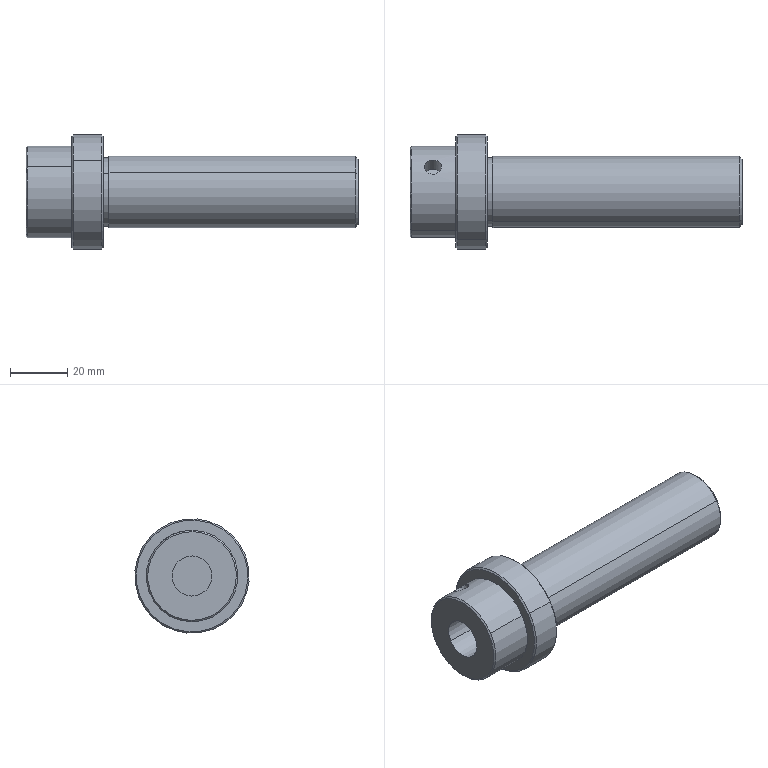Component | SolidWorks | 4-12-12ClampingAxisAssembly-1_4-12-3ClampingAxis-1 | 1 solid | 27 faces | box 116 x 40 x 40 mm | volume 68513 mm3 | cylinder 12 | cone 8 | plane 7 | commonest cylinder face diameters 6 x2 40 x2 32 x2 14 x2 25 x2 24 x2
build123d program:
from build123d import *

# Parameters (mm, degrees)
CHAMFER1_SIZE      = 1
CHAMFER2_SIZE      = 0.5
SKETCH2_R          = 3
CUT_EXTRUDE1_DEPTH = 6


with BuildPart() as part:
    # Sketch1 → Revolve1 (revolve)
    with BuildSketch(Plane(origin=(0, 0, 0), x_dir=(0, 0, -1), z_dir=(1, 0, 0)), mode=Mode.PRIVATE) as revolve1_sk:
        Polygon((0, 7), (0, 16), (16, 16), (16, 20), (27, 20), (27, 12), (29, 12), (29, 12.5), (116, 12.5), (116, 0), (10, 0), (10, 7), align=None)
    revolve(revolve1_sk.sketch.rotate(Axis((0, 0, 0), (0, 0, -1)), 90), axis=Axis((0, 0, 0), (0, 0, -1)))

    # Chamfer1
    chamfer1_edges = [part.edges().sort_by_distance(p)[0] for p in [
        (-12.5, 0, -116),
    ]]
    chamfer(chamfer1_edges, length=CHAMFER1_SIZE)

    # Chamfer2
    chamfer2_edges = [part.edges().sort_by_distance(p)[0] for p in [
        (-20, 0, -27),
        (-20, 0, -16),
        (-16, 0, 0),
    ]]
    chamfer(chamfer2_edges, length=CHAMFER2_SIZE)

    # Sketch2 → Cut-Extrude1 (cut)
    with BuildSketch(Plane(origin=(0, 16, 0), x_dir=(-1, 0, 0), z_dir=(0, 1, 0))):
        with Locations(Location((0, -8, 0), (0, 0, 90))):
            Circle(SKETCH2_R)
    extrude(amount=-CUT_EXTRUDE1_DEPTH, mode=Mode.SUBTRACT)


solid = part.part

# Placed as in the assembly
solid = solid.moved(Location((-152.809, -4.181, 0), (-166.184, -90, 137.125)))
STEP:
#1=COLOUR_RGB('',0.7922,0.8196,0.9333);
#2=FILL_AREA_STYLE_COLOUR('',#1);
#3=FILL_AREA_STYLE('',(#2));
#4=SURFACE_STYLE_FILL_AREA(#3);
#5=SURFACE_SIDE_STYLE('',(#4));
#6=SURFACE_STYLE_USAGE(.BOTH.,#5);
#7=PRESENTATION_STYLE_ASSIGNMENT((#6));
#8=CARTESIAN_POINT('',(-5.583,0.05163,0.329));
#9=VERTEX_POINT('',#8);
#10=CARTESIAN_POINT('',(-5.819,0.05163,0.329));
#11=VERTEX_POINT('',#10);
#12=CARTESIAN_POINT('',(-5.701,0.05163,0.329));
#13=DIRECTION('',(-0.,0.5492,0.8357));
#14=DIRECTION('',(-1.,-0.,0.));
#15=AXIS2_PLACEMENT_3D('',#12,#13,#14);
#16=CIRCLE('',#15,0.1181);
#17=EDGE_CURVE('',#9,#11,#16,.T.);
#18=ORIENTED_EDGE('',*,*,#17,.F.);
#19=CARTESIAN_POINT('',(-5.583,0.1814,0.5264));
#20=VERTEX_POINT('',#19);
#21=CARTESIAN_POINT('',(-5.583,0.05163,0.329));
#22=DIRECTION('',(-0.,0.5492,0.8357));
#23=VECTOR('',#22,39.37);
#24=LINE('',#21,#23);
#25=EDGE_CURVE('',#9,#20,#24,.T.);
#26=ORIENTED_EDGE('',*,*,#25,.T.);
#27=CARTESIAN_POINT('',(-5.819,0.1814,0.5264));
#28=VERTEX_POINT('',#27);
#29=CARTESIAN_POINT('',(-5.819,0.1814,0.5264));
#30=CARTESIAN_POINT('',(-5.819,0.1879,0.5221));
#31=CARTESIAN_POINT('',(-5.818,0.1943,0.5178));
#32=CARTESIAN_POINT('',(-5.815,0.2066,0.509));
#33=CARTESIAN_POINT('',(-5.813,0.2126,0.5045));
#34=CARTESIAN_POINT('',(-5.807,0.224,0.4958));
#35=CARTESIAN_POINT('',(-5.804,0.2293,0.4916));
#36=CARTESIAN_POINT('',(-5.795,0.2393,0.4834));
#37=CARTESIAN_POINT('',(-5.79,0.244,0.4795));
#38=CARTESIAN_POINT('',(-5.779,0.2523,0.4723));
#39=CARTESIAN_POINT('',(-5.773,0.2559,0.469));
#40=CARTESIAN_POINT('',(-5.76,0.2624,0.4631));
#41=CARTESIAN_POINT('',(-5.754,0.2651,0.4606));
#42=CARTESIAN_POINT('',(-5.739,0.2695,0.4565));
#43=CARTESIAN_POINT('',(-5.732,0.2712,0.4549));
#44=CARTESIAN_POINT('',(-5.717,0.2734,0.4527));
#45=CARTESIAN_POINT('',(-5.709,0.2739,0.4522));
#46=CARTESIAN_POINT('',(-5.693,0.2739,0.4522));
#47=CARTESIAN_POINT('',(-5.686,0.2734,0.4527));
#48=CARTESIAN_POINT('',(-5.67,0.2712,0.4549));
#49=CARTESIAN_POINT('',(-5.663,0.2695,0.4565));
#50=CARTESIAN_POINT('',(-5.649,0.2651,0.4606));
#51=CARTESIAN_POINT('',(-5.642,0.2624,0.4631));
#52=CARTESIAN_POINT('',(-5.629,0.256,0.469));
#53=CARTESIAN_POINT('',(-5.623,0.2523,0.4723));
#54=CARTESIAN_POINT('',(-5.612,0.2439,0.4795));
#55=CARTESIAN_POINT('',(-5.607,0.2393,0.4834));
#56=CARTESIAN_POINT('',(-5.599,0.2294,0.4915));
#57=CARTESIAN_POINT('',(-5.595,0.224,0.4958));
#58=CARTESIAN_POINT('',(-5.589,0.2126,0.5046));
#59=CARTESIAN_POINT('',(-5.587,0.2067,0.5089));
#60=CARTESIAN_POINT('',(-5.584,0.1943,0.5177));
#61=CARTESIAN_POINT('',(-5.583,0.1878,0.5222));
#62=CARTESIAN_POINT('',(-5.583,0.1814,0.5264));
#63=B_SPLINE_CURVE_WITH_KNOTS('',3,(#29,#30,#31,#32,#33,#34,#35,#36,#37,#38,#39,#40,#41,#42,#43,#44,#45,#46,#47,#48,#49,#50,#51,#52,#53,#54,#55,#56,#57,#58,#59,#60,#61,#62),.UNSPECIFIED.,.F.,.F.,(4,2,2,2,2,2,2,2,2,2,2,2,2,2,2,2,4),(0.,0.0005875,0.001175,0.001763,0.00235,0.002938,0.003525,0.004113,0.0047,0.005288,0.005875,0.006463,0.00705,0.007638,0.008225,0.008813,0.0094),.UNSPECIFIED.);
#64=EDGE_CURVE('',#28,#20,#63,.T.);
#65=ORIENTED_EDGE('',*,*,#64,.F.);
#66=CARTESIAN_POINT('',(-5.819,0.05163,0.329));
#67=DIRECTION('',(-0.,0.5492,0.8357));
#68=VECTOR('',#67,39.37);
#69=LINE('',#66,#68);
#70=EDGE_CURVE('',#11,#28,#69,.T.);
#71=ORIENTED_EDGE('',*,*,#70,.F.);
#72=EDGE_LOOP('',(#18,#26,#65,#71));
#73=FACE_OUTER_BOUND('',#72,.T.);
#74=CARTESIAN_POINT('',(-5.701,0.05163,0.329));
#75=DIRECTION('',(-0.,0.5492,0.8357));
#76=DIRECTION('',(-1.,-0.,0.));
#77=AXIS2_PLACEMENT_3D('',#74,#75,#76);
#78=CYLINDRICAL_SURFACE('',#77,0.1181);
#79=ADVANCED_FACE('',(#73),#78,.F.);
#80=CARTESIAN_POINT('',(-4.953,0.4769,-0.4217));
#81=VERTEX_POINT('',#80);
#82=CARTESIAN_POINT('',(-4.953,-0.8062,0.4217));
#83=VERTEX_POINT('',#82);
#84=CARTESIAN_POINT('',(-4.953,-0.1646,0.));
#85=DIRECTION('',(1.,0.,0.));
#86=DIRECTION('',(0.,-0.8357,0.5492));
#87=AXIS2_PLACEMENT_3D('',#84,#85,#86);
#88=CIRCLE('',#87,0.7677);
#89=EDGE_CURVE('',#81,#83,#88,.T.);
#90=ORIENTED_EDGE('',*,*,#89,.F.);
#91=CARTESIAN_POINT('',(-4.973,0.4934,-0.4325));
#92=VERTEX_POINT('',#91);
#93=CARTESIAN_POINT('',(-4.973,0.4934,-0.4325));
#94=DIRECTION('',(-0.7071,0.5909,-0.3884));
#95=VECTOR('',#94,39.37);
#96=LINE('',#93,#95);
#97=EDGE_CURVE('',#81,#92,#96,.T.);
#98=ORIENTED_EDGE('',*,*,#97,.T.);
#99=CARTESIAN_POINT('',(-4.973,-0.8226,0.4325));
#100=VERTEX_POINT('',#99);
#101=CARTESIAN_POINT('',(-4.973,-0.1646,0.));
#102=DIRECTION('',(-1.,-0.,-0.));
#103=DIRECTION('',(0.,-0.8357,0.5492));
#104=AXIS2_PLACEMENT_3D('',#101,#102,#103);
#105=CIRCLE('',#104,0.7874);
#106=EDGE_CURVE('',#100,#92,#105,.T.);
#107=ORIENTED_EDGE('',*,*,#106,.F.);
#108=CARTESIAN_POINT('',(-4.973,-0.8226,0.4325));
#109=DIRECTION('',(-0.7071,-0.5909,0.3884));
#110=VECTOR('',#109,39.37);
#111=LINE('',#108,#110);
#112=EDGE_CURVE('',#83,#100,#111,.T.);
#113=ORIENTED_EDGE('',*,*,#112,.F.);
#114=EDGE_LOOP('',(#90,#98,#107,#113));
#115=FACE_OUTER_BOUND('',#114,.T.);
#116=CARTESIAN_POINT('',(-4.973,-0.1646,0.));
#117=DIRECTION('',(-1.,-0.,-0.));
#118=DIRECTION('',(0.,-0.8357,0.5492));
#119=AXIS2_PLACEMENT_3D('',#116,#117,#118);
#120=CONICAL_SURFACE('',#119,0.7874,0.7854);
#121=ADVANCED_FACE('',(#115),#120,.T.);
#122=CARTESIAN_POINT('',(-5.386,-0.8062,0.4217));
#123=VERTEX_POINT('',#122);
#124=CARTESIAN_POINT('',(-5.386,0.4769,-0.4217));
#125=VERTEX_POINT('',#124);
#126=CARTESIAN_POINT('',(-5.386,-0.1646,0.));
#127=DIRECTION('',(-1.,-0.,-0.));
#128=DIRECTION('',(0.,0.8357,-0.5492));
#129=AXIS2_PLACEMENT_3D('',#126,#127,#128);
#130=CIRCLE('',#129,0.7677);
#131=EDGE_CURVE('',#123,#125,#130,.T.);
#132=ORIENTED_EDGE('',*,*,#131,.F.);
#133=CARTESIAN_POINT('',(-5.366,-0.8226,0.4325));
#134=VERTEX_POINT('',#133);
#135=CARTESIAN_POINT('',(-5.386,-0.8062,0.4217));
#136=DIRECTION('',(0.7071,-0.5909,0.3884));
#137=VECTOR('',#136,39.37);
#138=LINE('',#135,#137);
#139=EDGE_CURVE('',#123,#134,#138,.T.);
#140=ORIENTED_EDGE('',*,*,#139,.T.);
#141=CARTESIAN_POINT('',(-5.366,0.4934,-0.4325));
#142=VERTEX_POINT('',#141);
#143=CARTESIAN_POINT('',(-5.366,-0.1646,0.));
#144=DIRECTION('',(1.,0.,0.));
#145=DIRECTION('',(0.,0.8357,-0.5492));
#146=AXIS2_PLACEMENT_3D('',#143,#144,#145);
#147=CIRCLE('',#146,0.7874);
#148=EDGE_CURVE('',#142,#134,#147,.T.);
#149=ORIENTED_EDGE('',*,*,#148,.F.);
#150=CARTESIAN_POINT('',(-5.386,0.4769,-0.4217));
#151=DIRECTION('',(0.7071,0.5909,-0.3884));
#152=VECTOR('',#151,39.37);
#153=LINE('',#150,#152);
#154=EDGE_CURVE('',#125,#142,#153,.T.);
#155=ORIENTED_EDGE('',*,*,#154,.F.);
#156=EDGE_LOOP('',(#132,#140,#149,#155));
#157=FACE_OUTER_BOUND('',#156,.T.);
#158=CARTESIAN_POINT('',(-5.386,-0.1646,0.));
#159=DIRECTION('',(1.,0.,0.));
#160=DIRECTION('',(0.,0.8357,-0.5492));
#161=AXIS2_PLACEMENT_3D('',#158,#159,#160);
#162=CONICAL_SURFACE('',#161,0.7677,0.7854);
#163=ADVANCED_FACE('',(#157),#162,.T.);
#164=CARTESIAN_POINT('',(-6.016,-0.6746,0.3352));
#165=VERTEX_POINT('',#164);
#166=CARTESIAN_POINT('',(-6.016,0.3453,-0.3352));
#167=VERTEX_POINT('',#166);
#168=CARTESIAN_POINT('',(-6.016,-0.1646,-0.));
#169=DIRECTION('',(-1.,-0.,-0.));
#170=DIRECTION('',(0.,0.8357,-0.5492));
#171=AXIS2_PLACEMENT_3D('',#168,#169,#170);
#172=CIRCLE('',#171,0.6102);
#173=EDGE_CURVE('',#165,#167,#172,.T.);
#174=ORIENTED_EDGE('',*,*,#173,.F.);
#175=CARTESIAN_POINT('',(-5.996,-0.691,0.346));
#176=VERTEX_POINT('',#175);
#177=CARTESIAN_POINT('',(-6.016,-0.6746,0.3352));
#178=DIRECTION('',(0.7071,-0.5909,0.3884));
#179=VECTOR('',#178,39.37);
#180=LINE('',#177,#179);
#181=EDGE_CURVE('',#165,#176,#180,.T.);
#182=ORIENTED_EDGE('',*,*,#181,.T.);
#183=CARTESIAN_POINT('',(-5.996,0.3618,-0.346));
#184=VERTEX_POINT('',#183);
#185=CARTESIAN_POINT('',(-5.996,-0.1646,-0.));
#186=DIRECTION('',(1.,0.,0.));
#187=DIRECTION('',(0.,0.8357,-0.5492));
#188=AXIS2_PLACEMENT_3D('',#185,#186,#187);
#189=CIRCLE('',#188,0.6299);
#190=EDGE_CURVE('',#184,#176,#189,.T.);
#191=ORIENTED_EDGE('',*,*,#190,.F.);
#192=CARTESIAN_POINT('',(-6.016,0.3453,-0.3352));
#193=DIRECTION('',(0.7071,0.5909,-0.3884));
#194=VECTOR('',#193,39.37);
#195=LINE('',#192,#194);
#196=EDGE_CURVE('',#167,#184,#195,.T.);
#197=ORIENTED_EDGE('',*,*,#196,.F.);
#198=EDGE_LOOP('',(#174,#182,#191,#197));
#199=FACE_OUTER_BOUND('',#198,.T.);
#200=CARTESIAN_POINT('',(-6.016,-0.1646,-0.));
#201=DIRECTION('',(1.,0.,0.));
#202=DIRECTION('',(0.,0.8357,-0.5492));
#203=AXIS2_PLACEMENT_3D('',#200,#201,#202);
#204=CONICAL_SURFACE('',#203,0.6102,0.7854);
#205=ADVANCED_FACE('',(#199),#204,.T.);
#206=CARTESIAN_POINT('',(-1.449,0.2137,-0.2487));
#207=VERTEX_POINT('',#206);
#208=CARTESIAN_POINT('',(-1.449,-0.543,0.2487));
#209=VERTEX_POINT('',#208);
#210=CARTESIAN_POINT('',(-1.449,-0.1646,0.));
#211=DIRECTION('',(1.,0.,0.));
#212=DIRECTION('',(0.,-0.8357,0.5492));
#213=AXIS2_PLACEMENT_3D('',#210,#211,#212);
#214=CIRCLE('',#213,0.4528);
#215=EDGE_CURVE('',#207,#209,#214,.T.);
#216=ORIENTED_EDGE('',*,*,#215,.F.);
#217=CARTESIAN_POINT('',(-1.489,0.2466,-0.2703));
#218=VERTEX_POINT('',#217);
#219=CARTESIAN_POINT('',(-1.489,0.2466,-0.2703));
#220=DIRECTION('',(-0.7071,0.5909,-0.3884));
#221=VECTOR('',#220,39.37);
#222=LINE('',#219,#221);
#223=EDGE_CURVE('',#207,#218,#222,.T.);
#224=ORIENTED_EDGE('',*,*,#223,.T.);
#225=CARTESIAN_POINT('',(-1.489,-0.5759,0.2703));
#226=VERTEX_POINT('',#225);
#227=CARTESIAN_POINT('',(-1.489,-0.1646,0.));
#228=DIRECTION('',(-1.,-0.,-0.));
#229=DIRECTION('',(0.,-0.8357,0.5492));
#230=AXIS2_PLACEMENT_3D('',#227,#228,#229);
#231=CIRCLE('',#230,0.4921);
#232=EDGE_CURVE('',#226,#218,#231,.T.);
#233=ORIENTED_EDGE('',*,*,#232,.F.);
#234=CARTESIAN_POINT('',(-1.489,-0.5759,0.2703));
#235=DIRECTION('',(-0.7071,-0.5909,0.3884));
#236=VECTOR('',#235,39.37);
#237=LINE('',#234,#236);
#238=EDGE_CURVE('',#209,#226,#237,.T.);
#239=ORIENTED_EDGE('',*,*,#238,.F.);
#240=EDGE_LOOP('',(#216,#224,#233,#239));
#241=FACE_OUTER_BOUND('',#240,.T.);
#242=CARTESIAN_POINT('',(-1.489,-0.1646,0.));
#243=DIRECTION('',(-1.,-0.,-0.));
#244=DIRECTION('',(0.,-0.8357,0.5492));
#245=AXIS2_PLACEMENT_3D('',#242,#243,#244);
#246=CONICAL_SURFACE('',#245,0.4921,0.7854);
#247=ADVANCED_FACE('',(#241),#246,.T.);
#248=ORIENTED_EDGE('',*,*,#106,.T.);
#249=CARTESIAN_POINT('',(-6.016,0.4934,-0.4325));
#250=DIRECTION('',(-1.,-0.,-0.));
#251=VECTOR('',#250,39.37);
#252=LINE('',#249,#251);
#253=EDGE_CURVE('',#92,#142,#252,.T.);
#254=ORIENTED_EDGE('',*,*,#253,.T.);
#255=ORIENTED_EDGE('',*,*,#148,.T.);
#256=CARTESIAN_POINT('',(-6.016,-0.8226,0.4325));
#257=DIRECTION('',(-1.,-0.,-0.));
#258=VECTOR('',#257,39.37);
#259=LINE('',#256,#258);
#260=EDGE_CURVE('',#100,#134,#259,.T.);
#261=ORIENTED_EDGE('',*,*,#260,.F.);
#262=EDGE_LOOP('',(#248,#254,#255,#261));
#263=FACE_OUTER_BOUND('',#262,.T.);
#264=CARTESIAN_POINT('',(-6.016,-0.1646,-0.));
#265=DIRECTION('',(-1.,-0.,-0.));
#266=DIRECTION('',(0.,-0.8357,0.5492));
#267=AXIS2_PLACEMENT_3D('',#264,#265,#266);
#268=CYLINDRICAL_SURFACE('',#267,0.7874);
#269=ADVANCED_FACE('',(#263),#268,.T.);
#270=ORIENTED_EDGE('',*,*,#64,.T.);
#271=CARTESIAN_POINT('',(-5.583,0.1814,0.5264));
#272=CARTESIAN_POINT('',(-5.583,0.1749,0.5306));
#273=CARTESIAN_POINT('',(-5.584,0.1684,0.5347));
#274=CARTESIAN_POINT('',(-5.587,0.1553,0.5427));
#275=CARTESIAN_POINT('',(-5.589,0.1489,0.5464));
#276=CARTESIAN_POINT('',(-5.595,0.1365,0.5534));
#277=CARTESIAN_POINT('',(-5.599,0.1304,0.5566));
#278=CARTESIAN_POINT('',(-5.607,0.1189,0.5626));
#279=CARTESIAN_POINT('',(-5.612,0.1135,0.5652));
#280=CARTESIAN_POINT('',(-5.623,0.1036,0.57));
#281=CARTESIAN_POINT('',(-5.629,0.09905,0.5721));
#282=CARTESIAN_POINT('',(-5.642,0.09116,0.5757));
#283=CARTESIAN_POINT('',(-5.649,0.08778,0.5772));
#284=CARTESIAN_POINT('',(-5.663,0.08223,0.5796));
#285=CARTESIAN_POINT('',(-5.67,0.0801,0.5804));
#286=CARTESIAN_POINT('',(-5.686,0.07727,0.5816));
#287=CARTESIAN_POINT('',(-5.693,0.07654,0.5819));
#288=CARTESIAN_POINT('',(-5.709,0.07653,0.5819));
#289=CARTESIAN_POINT('',(-5.717,0.07724,0.5816));
#290=CARTESIAN_POINT('',(-5.732,0.08006,0.5805));
#291=CARTESIAN_POINT('',(-5.739,0.0822,0.5796));
#292=CARTESIAN_POINT('',(-5.753,0.08771,0.5772));
#293=CARTESIAN_POINT('',(-5.76,0.09108,0.5757));
#294=CARTESIAN_POINT('',(-5.773,0.09899,0.5721));
#295=CARTESIAN_POINT('',(-5.779,0.1035,0.57));
#296=CARTESIAN_POINT('',(-5.795,0.1183,0.5629));
#297=CARTESIAN_POINT('',(-5.804,0.1301,0.5569));
#298=CARTESIAN_POINT('',(-5.813,0.1488,0.5465));
#299=CARTESIAN_POINT('',(-5.815,0.1553,0.5427));
#300=CARTESIAN_POINT('',(-5.818,0.1683,0.5348));
#301=CARTESIAN_POINT('',(-5.819,0.1748,0.5307));
#302=CARTESIAN_POINT('',(-5.819,0.1814,0.5264));
#303=B_SPLINE_CURVE_WITH_KNOTS('',3,(#271,#272,#273,#274,#275,#276,#277,#278,#279,#280,#281,#282,#283,#284,#285,#286,#287,#288,#289,#290,#291,#292,#293,#294,#295,#296,#297,#298,#299,#300,#301,#302),.UNSPECIFIED.,.F.,.F.,(4,2,2,2,2,2,2,2,2,2,2,2,2,2,2,4),(0.0094,0.009988,0.01057,0.01116,0.01175,0.01234,0.01292,0.01351,0.0141,0.01469,0.01527,0.01586,0.01645,0.01762,0.01821,0.0188),.UNSPECIFIED.);
#304=EDGE_CURVE('',#20,#28,#303,.T.);
#305=ORIENTED_EDGE('',*,*,#304,.T.);
#306=EDGE_LOOP('',(#270,#305));
#307=FACE_BOUND('',#306,.T.);
#308=CARTESIAN_POINT('',(-5.386,-0.691,0.346));
#309=VERTEX_POINT('',#308);
#310=CARTESIAN_POINT('',(-5.386,0.3618,-0.346));
#311=VERTEX_POINT('',#310);
#312=CARTESIAN_POINT('',(-5.386,-0.1646,0.));
#313=DIRECTION('',(-1.,-0.,-0.));
#314=DIRECTION('',(0.,-0.8357,0.5492));
#315=AXIS2_PLACEMENT_3D('',#312,#313,#314);
#316=CIRCLE('',#315,0.6299);
#317=EDGE_CURVE('',#309,#311,#316,.T.);
#318=ORIENTED_EDGE('',*,*,#317,.T.);
#319=CARTESIAN_POINT('',(-6.016,0.3618,-0.346));
#320=DIRECTION('',(-1.,-0.,-0.));
#321=VECTOR('',#320,39.37);
#322=LINE('',#319,#321);
#323=EDGE_CURVE('',#311,#184,#322,.T.);
#324=ORIENTED_EDGE('',*,*,#323,.T.);
#325=ORIENTED_EDGE('',*,*,#190,.T.);
#326=CARTESIAN_POINT('',(-6.016,-0.691,0.346));
#327=DIRECTION('',(-1.,-0.,-0.));
#328=VECTOR('',#327,39.37);
#329=LINE('',#326,#328);
#330=EDGE_CURVE('',#309,#176,#329,.T.);
#331=ORIENTED_EDGE('',*,*,#330,.F.);
#332=EDGE_LOOP('',(#318,#324,#325,#331));
#333=FACE_OUTER_BOUND('',#332,.T.);
#334=CARTESIAN_POINT('',(-6.016,-0.1646,-0.));
#335=DIRECTION('',(-1.,-0.,-0.));
#336=DIRECTION('',(0.,-0.8357,0.5492));
#337=AXIS2_PLACEMENT_3D('',#334,#335,#336);
#338=CYLINDRICAL_SURFACE('',#337,0.6299);
#339=ADVANCED_FACE('',(#307,#333),#338,.T.);
#340=CARTESIAN_POINT('',(-5.622,0.0657,-0.1514));
#341=VERTEX_POINT('',#340);
#342=CARTESIAN_POINT('',(-5.622,-0.3949,0.1514));
#343=VERTEX_POINT('',#342);
#344=CARTESIAN_POINT('',(-5.622,-0.1646,-0.));
#345=DIRECTION('',(-1.,-0.,-0.));
#346=DIRECTION('',(0.,-0.8357,0.5492));
#347=AXIS2_PLACEMENT_3D('',#344,#345,#346);
#348=CIRCLE('',#347,0.2756);
#349=EDGE_CURVE('',#341,#343,#348,.T.);
#350=ORIENTED_EDGE('',*,*,#349,.F.);
#351=CARTESIAN_POINT('',(-6.016,0.0657,-0.1514));
#352=VERTEX_POINT('',#351);
#353=CARTESIAN_POINT('',(-6.016,0.0657,-0.1514));
#354=DIRECTION('',(-1.,-0.,-0.));
#355=VECTOR('',#354,39.37);
#356=LINE('',#353,#355);
#357=EDGE_CURVE('',#341,#352,#356,.T.);
#358=ORIENTED_EDGE('',*,*,#357,.T.);
#359=CARTESIAN_POINT('',(-6.016,-0.3949,0.1514));
#360=VERTEX_POINT('',#359);
#361=CARTESIAN_POINT('',(-6.016,-0.1646,-0.));
#362=DIRECTION('',(-1.,-0.,-0.));
#363=DIRECTION('',(0.,-0.8357,0.5492));
#364=AXIS2_PLACEMENT_3D('',#361,#362,#363);
#365=CIRCLE('',#364,0.2756);
#366=EDGE_CURVE('',#352,#360,#365,.T.);
#367=ORIENTED_EDGE('',*,*,#366,.T.);
#368=CARTESIAN_POINT('',(-6.016,-0.3949,0.1514));
#369=DIRECTION('',(-1.,-0.,-0.));
#370=VECTOR('',#369,39.37);
#371=LINE('',#368,#370);
#372=EDGE_CURVE('',#343,#360,#371,.T.);
#373=ORIENTED_EDGE('',*,*,#372,.F.);
#374=EDGE_LOOP('',(#350,#358,#367,#373));
#375=FACE_OUTER_BOUND('',#374,.T.);
#376=CARTESIAN_POINT('',(-6.016,-0.1646,-0.));
#377=DIRECTION('',(-1.,-0.,-0.));
#378=DIRECTION('',(0.,-0.8357,0.5492));
#379=AXIS2_PLACEMENT_3D('',#376,#377,#378);
#380=CYLINDRICAL_SURFACE('',#379,0.2756);
#381=ADVANCED_FACE('',(#375),#380,.F.);
#382=ORIENTED_EDGE('',*,*,#232,.T.);
#383=CARTESIAN_POINT('',(-4.874,0.2466,-0.2703));
#384=VERTEX_POINT('',#383);
#385=CARTESIAN_POINT('',(-6.016,0.2466,-0.2703));
#386=DIRECTION('',(-1.,-0.,-0.));
#387=VECTOR('',#386,39.37);
#388=LINE('',#385,#387);
#389=EDGE_CURVE('',#218,#384,#388,.T.);
#390=ORIENTED_EDGE('',*,*,#389,.T.);
#391=CARTESIAN_POINT('',(-4.874,-0.5759,0.2703));
#392=VERTEX_POINT('',#391);
#393=CARTESIAN_POINT('',(-4.874,-0.1646,0.));
#394=DIRECTION('',(-1.,-0.,-0.));
#395=DIRECTION('',(0.,-0.8357,0.5492));
#396=AXIS2_PLACEMENT_3D('',#393,#394,#395);
#397=CIRCLE('',#396,0.4921);
#398=EDGE_CURVE('',#392,#384,#397,.T.);
#399=ORIENTED_EDGE('',*,*,#398,.F.);
#400=CARTESIAN_POINT('',(-6.016,-0.5759,0.2703));
#401=DIRECTION('',(-1.,-0.,-0.));
#402=VECTOR('',#401,39.37);
#403=LINE('',#400,#402);
#404=EDGE_CURVE('',#226,#392,#403,.T.);
#405=ORIENTED_EDGE('',*,*,#404,.F.);
#406=EDGE_LOOP('',(#382,#390,#399,#405));
#407=FACE_OUTER_BOUND('',#406,.T.);
#408=CARTESIAN_POINT('',(-6.016,-0.1646,-0.));
#409=DIRECTION('',(-1.,-0.,-0.));
#410=DIRECTION('',(0.,-0.8357,0.5492));
#411=AXIS2_PLACEMENT_3D('',#408,#409,#410);
#412=CYLINDRICAL_SURFACE('',#411,0.4921);
#413=ADVANCED_FACE('',(#407),#412,.T.);
#414=CARTESIAN_POINT('',(-4.874,-0.5594,0.2595));
#415=VERTEX_POINT('',#414);
#416=CARTESIAN_POINT('',(-4.874,0.2302,-0.2595));
#417=VERTEX_POINT('',#416);
#418=CARTESIAN_POINT('',(-4.874,-0.1646,0.));
#419=DIRECTION('',(-1.,-0.,-0.));
#420=DIRECTION('',(0.,-0.8357,0.5492));
#421=AXIS2_PLACEMENT_3D('',#418,#419,#420);
#422=CIRCLE('',#421,0.4724);
#423=EDGE_CURVE('',#415,#417,#422,.T.);
#424=ORIENTED_EDGE('',*,*,#423,.T.);
#425=CARTESIAN_POINT('',(-4.953,0.2302,-0.2595));
#426=VERTEX_POINT('',#425);
#427=CARTESIAN_POINT('',(-6.016,0.2302,-0.2595));
#428=DIRECTION('',(-1.,-0.,-0.));
#429=VECTOR('',#428,39.37);
#430=LINE('',#427,#429);
#431=EDGE_CURVE('',#417,#426,#430,.T.);
#432=ORIENTED_EDGE('',*,*,#431,.T.);
#433=CARTESIAN_POINT('',(-4.953,-0.5594,0.2595));
#434=VERTEX_POINT('',#433);
#435=CARTESIAN_POINT('',(-4.953,-0.1646,0.));
#436=DIRECTION('',(-1.,-0.,-0.));
#437=DIRECTION('',(0.,-0.8357,0.5492));
#438=AXIS2_PLACEMENT_3D('',#435,#436,#437);
#439=CIRCLE('',#438,0.4724);
#440=EDGE_CURVE('',#434,#426,#439,.T.);
#441=ORIENTED_EDGE('',*,*,#440,.F.);
#442=CARTESIAN_POINT('',(-6.016,-0.5594,0.2595));
#443=DIRECTION('',(-1.,-0.,-0.));
#444=VECTOR('',#443,39.37);
#445=LINE('',#442,#444);
#446=EDGE_CURVE('',#415,#434,#445,.T.);
#447=ORIENTED_EDGE('',*,*,#446,.F.);
#448=EDGE_LOOP('',(#424,#432,#441,#447));
#449=FACE_OUTER_BOUND('',#448,.T.);
#450=CARTESIAN_POINT('',(-6.016,-0.1646,-0.));
#451=DIRECTION('',(-1.,-0.,-0.));
#452=DIRECTION('',(0.,-0.8357,0.5492));
#453=AXIS2_PLACEMENT_3D('',#450,#451,#452);
#454=CYLINDRICAL_SURFACE('',#453,0.4724);
#455=ADVANCED_FACE('',(#449),#454,.T.);
#456=CARTESIAN_POINT('',(-4.953,-0.1646,0.));
#457=DIRECTION('',(1.,0.,0.));
#458=DIRECTION('',(0.,-0.8357,0.5492));
#459=AXIS2_PLACEMENT_3D('',#456,#457,#458);
#460=CIRCLE('',#459,0.7677);
#461=EDGE_CURVE('',#83,#81,#460,.T.);
#462=ORIENTED_EDGE('',*,*,#461,.T.);
#463=ORIENTED_EDGE('',*,*,#89,.T.);
#464=EDGE_LOOP('',(#462,#463));
#465=FACE_OUTER_BOUND('',#464,.T.);
#466=ORIENTED_EDGE('',*,*,#440,.T.);
#467=CARTESIAN_POINT('',(-4.953,-0.1646,0.));
#468=DIRECTION('',(-1.,-0.,-0.));
#469=DIRECTION('',(0.,-0.8357,0.5492));
#470=AXIS2_PLACEMENT_3D('',#467,#468,#469);
#471=CIRCLE('',#470,0.4724);
#472=EDGE_CURVE('',#426,#434,#471,.T.);
#473=ORIENTED_EDGE('',*,*,#472,.T.);
#474=EDGE_LOOP('',(#466,#473));
#475=FACE_BOUND('',#474,.T.);
#476=CARTESIAN_POINT('',(-4.953,0.2679,0.658));
#477=DIRECTION('',(-1.,-0.,-0.));
#478=DIRECTION('',(0.,-0.8357,0.5492));
#479=AXIS2_PLACEMENT_3D('',#476,#477,#478);
#480=PLANE('',#479);
#481=ADVANCED_FACE('',(#465,#475),#480,.F.);
#482=ORIENTED_EDGE('',*,*,#431,.F.);
#483=CARTESIAN_POINT('',(-4.874,-0.1646,0.));
#484=DIRECTION('',(-1.,-0.,-0.));
#485=DIRECTION('',(0.,-0.8357,0.5492));
#486=AXIS2_PLACEMENT_3D('',#483,#484,#485);
#487=CIRCLE('',#486,0.4724);
#488=EDGE_CURVE('',#417,#415,#487,.T.);
#489=ORIENTED_EDGE('',*,*,#488,.T.);
#490=ORIENTED_EDGE('',*,*,#446,.T.);
#491=ORIENTED_EDGE('',*,*,#472,.F.);
#492=EDGE_LOOP('',(#482,#489,#490,#491));
#493=FACE_OUTER_BOUND('',#492,.T.);
#494=CARTESIAN_POINT('',(-6.016,-0.1646,-0.));
#495=DIRECTION('',(-1.,-0.,-0.));
#496=DIRECTION('',(0.,-0.8357,0.5492));
#497=AXIS2_PLACEMENT_3D('',#494,#495,#496);
#498=CYLINDRICAL_SURFACE('',#497,0.4724);
#499=ADVANCED_FACE('',(#493),#498,.T.);
#500=ORIENTED_EDGE('',*,*,#423,.F.);
#501=ORIENTED_EDGE('',*,*,#488,.F.);
#502=EDGE_LOOP('',(#500,#501));
#503=FACE_BOUND('',#502,.T.);
#504=ORIENTED_EDGE('',*,*,#398,.T.);
#505=CARTESIAN_POINT('',(-4.874,-0.1646,0.));
#506=DIRECTION('',(-1.,-0.,-0.));
#507=DIRECTION('',(0.,-0.8357,0.5492));
#508=AXIS2_PLACEMENT_3D('',#505,#506,#507);
#509=CIRCLE('',#508,0.4921);
#510=EDGE_CURVE('',#384,#392,#509,.T.);
#511=ORIENTED_EDGE('',*,*,#510,.T.);
#512=EDGE_LOOP('',(#504,#511));
#513=FACE_OUTER_BOUND('',#512,.T.);
#514=CARTESIAN_POINT('',(-4.874,0.09488,0.3948));
#515=DIRECTION('',(1.,0.,0.));
#516=DIRECTION('',(-0.,0.8357,-0.5492));
#517=AXIS2_PLACEMENT_3D('',#514,#515,#516);
#518=PLANE('',#517);
#519=ADVANCED_FACE('',(#503,#513),#518,.F.);
#520=ORIENTED_EDGE('',*,*,#389,.F.);
#521=CARTESIAN_POINT('',(-1.489,-0.1646,0.));
#522=DIRECTION('',(-1.,-0.,-0.));
#523=DIRECTION('',(0.,-0.8357,0.5492));
#524=AXIS2_PLACEMENT_3D('',#521,#522,#523);
#525=CIRCLE('',#524,0.4921);
#526=EDGE_CURVE('',#218,#226,#525,.T.);
#527=ORIENTED_EDGE('',*,*,#526,.T.);
#528=ORIENTED_EDGE('',*,*,#404,.T.);
#529=ORIENTED_EDGE('',*,*,#510,.F.);
#530=EDGE_LOOP('',(#520,#527,#528,#529));
#531=FACE_OUTER_BOUND('',#530,.T.);
#532=CARTESIAN_POINT('',(-6.016,-0.1646,-0.));
#533=DIRECTION('',(-1.,-0.,-0.));
#534=DIRECTION('',(0.,-0.8357,0.5492));
#535=AXIS2_PLACEMENT_3D('',#532,#533,#534);
#536=CYLINDRICAL_SURFACE('',#535,0.4921);
#537=ADVANCED_FACE('',(#531),#536,.T.);
#538=CARTESIAN_POINT('',(-1.449,-0.1646,0.));
#539=DIRECTION('',(1.,0.,0.));
#540=DIRECTION('',(0.,-0.8357,0.5492));
#541=AXIS2_PLACEMENT_3D('',#538,#539,#540);
#542=CIRCLE('',#541,0.4528);
#543=EDGE_CURVE('',#209,#207,#542,.T.);
#544=ORIENTED_EDGE('',*,*,#543,.T.);
#545=ORIENTED_EDGE('',*,*,#215,.T.);
#546=EDGE_LOOP('',(#544,#545));
#547=FACE_OUTER_BOUND('',#546,.T.);
#548=CARTESIAN_POINT('',(-1.449,0.1057,0.4113));
#549=DIRECTION('',(-1.,-0.,-0.));
#550=DIRECTION('',(0.,-0.8357,0.5492));
#551=AXIS2_PLACEMENT_3D('',#548,#549,#550);
#552=PLANE('',#551);
#553=ADVANCED_FACE('',(#547),#552,.F.);
#554=CARTESIAN_POINT('',(-5.622,-0.1646,-0.));
#555=DIRECTION('',(-1.,-0.,-0.));
#556=DIRECTION('',(0.,-0.8357,0.5492));
#557=AXIS2_PLACEMENT_3D('',#554,#555,#556);
#558=CIRCLE('',#557,0.2756);
#559=EDGE_CURVE('',#343,#341,#558,.T.);
#560=ORIENTED_EDGE('',*,*,#559,.T.);
#561=ORIENTED_EDGE('',*,*,#349,.T.);
#562=EDGE_LOOP('',(#560,#561));
#563=FACE_OUTER_BOUND('',#562,.T.);
#564=CARTESIAN_POINT('',(-5.622,-0.01324,0.2303));
#565=DIRECTION('',(1.,0.,0.));
#566=DIRECTION('',(-0.,0.8357,-0.5492));
#567=AXIS2_PLACEMENT_3D('',#564,#565,#566);
#568=PLANE('',#567);
#569=ADVANCED_FACE('',(#563),#568,.F.);
#570=ORIENTED_EDGE('',*,*,#357,.F.);
#571=ORIENTED_EDGE('',*,*,#559,.F.);
#572=ORIENTED_EDGE('',*,*,#372,.T.);
#573=CARTESIAN_POINT('',(-6.016,-0.1646,-0.));
#574=DIRECTION('',(-1.,-0.,-0.));
#575=DIRECTION('',(0.,-0.8357,0.5492));
#576=AXIS2_PLACEMENT_3D('',#573,#574,#575);
#577=CIRCLE('',#576,0.2756);
#578=EDGE_CURVE('',#360,#352,#577,.T.);
#579=ORIENTED_EDGE('',*,*,#578,.T.);
#580=EDGE_LOOP('',(#570,#571,#572,#579));
#581=FACE_OUTER_BOUND('',#580,.T.);
#582=CARTESIAN_POINT('',(-6.016,-0.1646,-0.));
#583=DIRECTION('',(-1.,-0.,-0.));
#584=DIRECTION('',(0.,-0.8357,0.5492));
#585=AXIS2_PLACEMENT_3D('',#582,#583,#584);
#586=CYLINDRICAL_SURFACE('',#585,0.2756);
#587=ADVANCED_FACE('',(#581),#586,.F.);
#588=CARTESIAN_POINT('',(-6.016,-0.1646,-0.));
#589=DIRECTION('',(-1.,-0.,-0.));
#590=DIRECTION('',(0.,0.8357,-0.5492));
#591=AXIS2_PLACEMENT_3D('',#588,#589,#590);
#592=CIRCLE('',#591,0.6102);
#593=EDGE_CURVE('',#167,#165,#592,.T.);
#594=ORIENTED_EDGE('',*,*,#593,.T.);
#595=ORIENTED_EDGE('',*,*,#173,.T.);
#596=EDGE_LOOP('',(#594,#595));
#597=FACE_OUTER_BOUND('',#596,.T.);
#598=ORIENTED_EDGE('',*,*,#578,.F.);
#599=ORIENTED_EDGE('',*,*,#366,.F.);
#600=EDGE_LOOP('',(#598,#599));
#601=FACE_BOUND('',#600,.T.);
#602=CARTESIAN_POINT('',(-6.016,-0.01324,0.2303));
#603=DIRECTION('',(1.,0.,0.));
#604=DIRECTION('',(-0.,0.8357,-0.5492));
#605=AXIS2_PLACEMENT_3D('',#602,#603,#604);
#606=PLANE('',#605);
#607=ADVANCED_FACE('',(#597,#601),#606,.F.);
#608=ORIENTED_EDGE('',*,*,#323,.F.);
#609=CARTESIAN_POINT('',(-5.386,-0.1646,0.));
#610=DIRECTION('',(-1.,-0.,-0.));
#611=DIRECTION('',(0.,-0.8357,0.5492));
#612=AXIS2_PLACEMENT_3D('',#609,#610,#611);
#613=CIRCLE('',#612,0.6299);
#614=EDGE_CURVE('',#311,#309,#613,.T.);
#615=ORIENTED_EDGE('',*,*,#614,.T.);
#616=ORIENTED_EDGE('',*,*,#330,.T.);
#617=CARTESIAN_POINT('',(-5.996,-0.1646,-0.));
#618=DIRECTION('',(1.,0.,0.));
#619=DIRECTION('',(0.,0.8357,-0.5492));
#620=AXIS2_PLACEMENT_3D('',#617,#618,#619);
#621=CIRCLE('',#620,0.6299);
#622=EDGE_CURVE('',#176,#184,#621,.T.);
#623=ORIENTED_EDGE('',*,*,#622,.T.);
#624=EDGE_LOOP('',(#608,#615,#616,#623));
#625=FACE_OUTER_BOUND('',#624,.T.);
#626=CARTESIAN_POINT('',(-6.016,-0.1646,-0.));
#627=DIRECTION('',(-1.,-0.,-0.));
#628=DIRECTION('',(0.,-0.8357,0.5492));
#629=AXIS2_PLACEMENT_3D('',#626,#627,#628);
#630=CYLINDRICAL_SURFACE('',#629,0.6299);
#631=ADVANCED_FACE('',(#625),#630,.T.);
#632=CARTESIAN_POINT('',(-5.386,-0.1646,0.));
#633=DIRECTION('',(-1.,-0.,-0.));
#634=DIRECTION('',(0.,0.8357,-0.5492));
#635=AXIS2_PLACEMENT_3D('',#632,#633,#634);
#636=CIRCLE('',#635,0.7677);
#637=EDGE_CURVE('',#125,#123,#636,.T.);
#638=ORIENTED_EDGE('',*,*,#637,.T.);
#639=ORIENTED_EDGE('',*,*,#131,.T.);
#640=EDGE_LOOP('',(#638,#639));
#641=FACE_OUTER_BOUND('',#640,.T.);
#642=ORIENTED_EDGE('',*,*,#317,.F.);
#643=ORIENTED_EDGE('',*,*,#614,.F.);
#644=EDGE_LOOP('',(#642,#643));
#645=FACE_BOUND('',#644,.T.);
#646=CARTESIAN_POINT('',(-5.386,0.1814,0.5264));
#647=DIRECTION('',(1.,0.,0.));
#648=DIRECTION('',(-0.,0.8357,-0.5492));
#649=AXIS2_PLACEMENT_3D('',#646,#647,#648);
#650=PLANE('',#649);
#651=ADVANCED_FACE('',(#641,#645),#650,.F.);
#652=ORIENTED_EDGE('',*,*,#253,.F.);
#653=CARTESIAN_POINT('',(-4.973,-0.1646,0.));
#654=DIRECTION('',(-1.,-0.,-0.));
#655=DIRECTION('',(0.,-0.8357,0.5492));
#656=AXIS2_PLACEMENT_3D('',#653,#654,#655);
#657=CIRCLE('',#656,0.7874);
#658=EDGE_CURVE('',#92,#100,#657,.T.);
#659=ORIENTED_EDGE('',*,*,#658,.T.);
#660=ORIENTED_EDGE('',*,*,#260,.T.);
#661=CARTESIAN_POINT('',(-5.366,-0.1646,0.));
#662=DIRECTION('',(1.,0.,0.));
#663=DIRECTION('',(0.,0.8357,-0.5492));
#664=AXIS2_PLACEMENT_3D('',#661,#662,#663);
#665=CIRCLE('',#664,0.7874);
#666=EDGE_CURVE('',#134,#142,#665,.T.);
#667=ORIENTED_EDGE('',*,*,#666,.T.);
#668=EDGE_LOOP('',(#652,#659,#660,#667));
#669=FACE_OUTER_BOUND('',#668,.T.);
#670=CARTESIAN_POINT('',(-6.016,-0.1646,-0.));
#671=DIRECTION('',(-1.,-0.,-0.));
#672=DIRECTION('',(0.,-0.8357,0.5492));
#673=AXIS2_PLACEMENT_3D('',#670,#671,#672);
#674=CYLINDRICAL_SURFACE('',#673,0.7874);
#675=ADVANCED_FACE('',(#669),#674,.T.);
#676=ORIENTED_EDGE('',*,*,#223,.F.);
#677=ORIENTED_EDGE('',*,*,#543,.F.);
#678=ORIENTED_EDGE('',*,*,#238,.T.);
#679=ORIENTED_EDGE('',*,*,#526,.F.);
#680=EDGE_LOOP('',(#676,#677,#678,#679));
#681=FACE_OUTER_BOUND('',#680,.T.);
#682=CARTESIAN_POINT('',(-1.489,-0.1646,0.));
#683=DIRECTION('',(-1.,-0.,-0.));
#684=DIRECTION('',(0.,-0.8357,0.5492));
#685=AXIS2_PLACEMENT_3D('',#682,#683,#684);
#686=CONICAL_SURFACE('',#685,0.4921,0.7854);
#687=ADVANCED_FACE('',(#681),#686,.T.);
#688=ORIENTED_EDGE('',*,*,#181,.F.);
#689=ORIENTED_EDGE('',*,*,#593,.F.);
#690=ORIENTED_EDGE('',*,*,#196,.T.);
#691=ORIENTED_EDGE('',*,*,#622,.F.);
#692=EDGE_LOOP('',(#688,#689,#690,#691));
#693=FACE_OUTER_BOUND('',#692,.T.);
#694=CARTESIAN_POINT('',(-6.016,-0.1646,-0.));
#695=DIRECTION('',(1.,0.,0.));
#696=DIRECTION('',(0.,0.8357,-0.5492));
#697=AXIS2_PLACEMENT_3D('',#694,#695,#696);
#698=CONICAL_SURFACE('',#697,0.6102,0.7854);
#699=ADVANCED_FACE('',(#693),#698,.T.);
#700=ORIENTED_EDGE('',*,*,#139,.F.);
#701=ORIENTED_EDGE('',*,*,#637,.F.);
#702=ORIENTED_EDGE('',*,*,#154,.T.);
#703=ORIENTED_EDGE('',*,*,#666,.F.);
#704=EDGE_LOOP('',(#700,#701,#702,#703));
#705=FACE_OUTER_BOUND('',#704,.T.);
#706=CARTESIAN_POINT('',(-5.386,-0.1646,0.));
#707=DIRECTION('',(1.,0.,0.));
#708=DIRECTION('',(0.,0.8357,-0.5492));
#709=AXIS2_PLACEMENT_3D('',#706,#707,#708);
#710=CONICAL_SURFACE('',#709,0.7677,0.7854);
#711=ADVANCED_FACE('',(#705),#710,.T.);
#712=ORIENTED_EDGE('',*,*,#97,.F.);
#713=ORIENTED_EDGE('',*,*,#461,.F.);
#714=ORIENTED_EDGE('',*,*,#112,.T.);
#715=ORIENTED_EDGE('',*,*,#658,.F.);
#716=EDGE_LOOP('',(#712,#713,#714,#715));
#717=FACE_OUTER_BOUND('',#716,.T.);
#718=CARTESIAN_POINT('',(-4.973,-0.1646,0.));
#719=DIRECTION('',(-1.,-0.,-0.));
#720=DIRECTION('',(0.,-0.8357,0.5492));
#721=AXIS2_PLACEMENT_3D('',#718,#719,#720);
#722=CONICAL_SURFACE('',#721,0.7874,0.7854);
#723=ADVANCED_FACE('',(#717),#722,.T.);
#724=ORIENTED_EDGE('',*,*,#25,.F.);
#725=CARTESIAN_POINT('',(-5.701,0.05163,0.329));
#726=DIRECTION('',(-0.,0.5492,0.8357));
#727=DIRECTION('',(-1.,-0.,0.));
#728=AXIS2_PLACEMENT_3D('',#725,#726,#727);
#729=CIRCLE('',#728,0.1181);
#730=EDGE_CURVE('',#11,#9,#729,.T.);
#731=ORIENTED_EDGE('',*,*,#730,.F.);
#732=ORIENTED_EDGE('',*,*,#70,.T.);
#733=ORIENTED_EDGE('',*,*,#304,.F.);
#734=EDGE_LOOP('',(#724,#731,#732,#733));
#735=FACE_OUTER_BOUND('',#734,.T.);
#736=CARTESIAN_POINT('',(-5.701,0.05163,0.329));
#737=DIRECTION('',(-0.,0.5492,0.8357));
#738=DIRECTION('',(-1.,-0.,0.));
#739=AXIS2_PLACEMENT_3D('',#736,#737,#738);
#740=CYLINDRICAL_SURFACE('',#739,0.1181);
#741=ADVANCED_FACE('',(#735),#740,.F.);
#742=ORIENTED_EDGE('',*,*,#730,.T.);
#743=ORIENTED_EDGE('',*,*,#17,.T.);
#744=EDGE_LOOP('',(#742,#743));
#745=FACE_OUTER_BOUND('',#744,.T.);
#746=CARTESIAN_POINT('',(-5.701,0.05163,0.329));
#747=DIRECTION('',(-0.,0.5492,0.8357));
#748=DIRECTION('',(-1.,-0.,-0.));
#749=AXIS2_PLACEMENT_3D('',#746,#747,#748);
#750=PLANE('',#749);
#751=ADVANCED_FACE('',(#745),#750,.T.);
#752=CLOSED_SHELL('',(#79,#121,#163,#205,#247,#269,#339,#381,#413,#455,#481,#499,#519,#537,#553,#569,#587,#607,#631,#651,#675,#687,#699,#711,#723,#741,#751));
#753=MANIFOLD_SOLID_BREP('',#752);
#754=STYLED_ITEM('',(#7),#753);
#755=(LENGTH_UNIT()NAMED_UNIT(*)SI_UNIT($,.METRE.));
#756=LENGTH_MEASURE_WITH_UNIT(LENGTH_MEASURE(0.0254),#755);
#757=DIMENSIONAL_EXPONENTS(1.,0.,0.,0.,0.,0.,0.);
#758=(CONVERSION_BASED_UNIT('',#756)LENGTH_UNIT()NAMED_UNIT(#757));
#759=UNCERTAINTY_MEASURE_WITH_UNIT(LENGTH_MEASURE(0.00001),#758,'','');
#760=(NAMED_UNIT(*)PLANE_ANGLE_UNIT()SI_UNIT($,.RADIAN.));
#761=(NAMED_UNIT(*)SI_UNIT($,.STERADIAN.)SOLID_ANGLE_UNIT());
#762=(GEOMETRIC_REPRESENTATION_CONTEXT(3)GLOBAL_UNCERTAINTY_ASSIGNED_CONTEXT((#759))GLOBAL_UNIT_ASSIGNED_CONTEXT((#758,#760,#761))REPRESENTATION_CONTEXT('',''));
#763=MECHANICAL_DESIGN_GEOMETRIC_PRESENTATION_REPRESENTATION('',(#754),#762);
#764=PRESENTATION_LAYER_ASSIGNMENT('','',(#754));
#765=CARTESIAN_POINT('',(0.,0.,0.));
#766=DIRECTION('',(0.,0.,1.));
#767=DIRECTION('',(1.,0.,0.));
#768=AXIS2_PLACEMENT_3D('',#765,#766,#767);
#769=(LENGTH_UNIT()NAMED_UNIT(*)SI_UNIT($,.METRE.));
#770=LENGTH_MEASURE_WITH_UNIT(LENGTH_MEASURE(0.0254),#769);
#771=DIMENSIONAL_EXPONENTS(1.,0.,0.,0.,0.,0.,0.);
#772=(CONVERSION_BASED_UNIT('',#770)LENGTH_UNIT()NAMED_UNIT(#771));
#773=UNCERTAINTY_MEASURE_WITH_UNIT(LENGTH_MEASURE(0.00001),#772,'','');
#774=(NAMED_UNIT(*)PLANE_ANGLE_UNIT()SI_UNIT($,.RADIAN.));
#775=(NAMED_UNIT(*)SI_UNIT($,.STERADIAN.)SOLID_ANGLE_UNIT());
#776=(GEOMETRIC_REPRESENTATION_CONTEXT(3)GLOBAL_UNCERTAINTY_ASSIGNED_CONTEXT((#773))GLOBAL_UNIT_ASSIGNED_CONTEXT((#772,#774,#775))REPRESENTATION_CONTEXT('',''));
#777=ADVANCED_BREP_SHAPE_REPRESENTATION('',(#753,#768),#776);